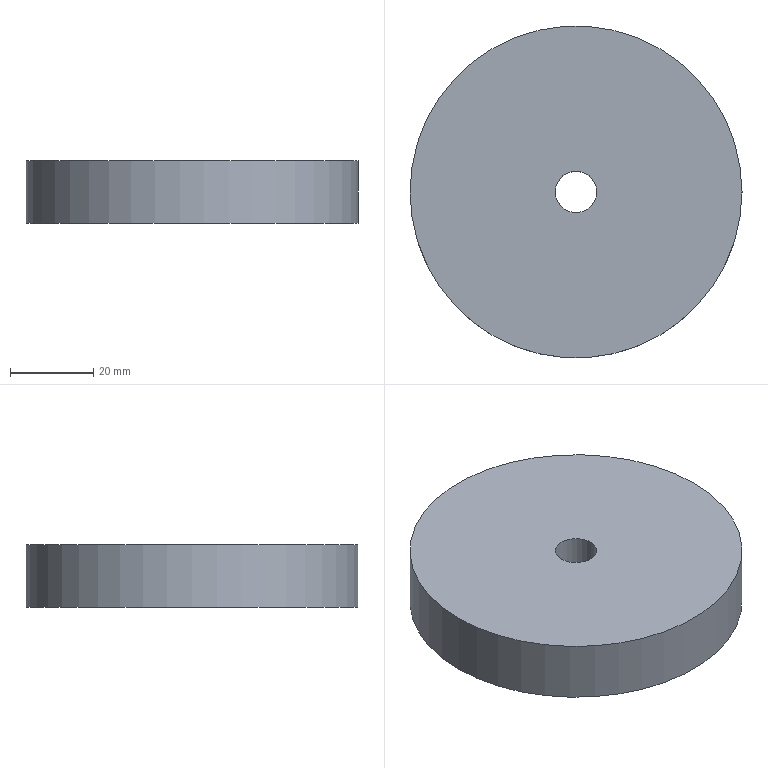Component | NX | CH3404_10-7 | 1 solid | 4 faces | box 80 x 80 x 15 mm | volume 74220 mm3 | cylinder 2 | plane 2 | commonest cylinder face diameters 80 x1 10 x1
STEP:
#1=CARTESIAN_POINT('',(0.,0.,0.));
#2=DIRECTION('',(0.,0.,1.));
#3=DIRECTION('',(1.,0.,0.));
#4=AXIS2_PLACEMENT_3D('',#1,#2,#3);
#5=CARTESIAN_POINT('',(40.,0.,202.));
#6=VERTEX_POINT('',#5);
#7=CARTESIAN_POINT('',(0.,0.,202.));
#8=DIRECTION('',(0.,0.,1.));
#9=DIRECTION('',(1.,0.,0.));
#10=AXIS2_PLACEMENT_3D('',#7,#8,#9);
#11=CIRCLE('',#10,40.);
#12=CARTESIAN_POINT('',(0.,0.,202.));
#13=DIRECTION('',(0.,0.,-1.));
#14=DIRECTION('',(-1.,0.,0.));
#15=AXIS2_PLACEMENT_3D('',#12,#13,#14);
#16=CYLINDRICAL_SURFACE('',#15,40.);
#17=CARTESIAN_POINT('',(9.425,0.));
#18=DIRECTION('',(-1.,0.));
#19=VECTOR('',#18,1.);
#20=LINE('',#17,#19);
#21=(GEOMETRIC_REPRESENTATION_CONTEXT(2)PARAMETRIC_REPRESENTATION_CONTEXT()REPRESENTATION_CONTEXT('',''));
#22=DEFINITIONAL_REPRESENTATION('',(#20),#21);
#23=PCURVE('',#16,#22);
#24=CARTESIAN_POINT('',(0.,0.,202.));
#25=DIRECTION('',(0.,0.,1.));
#26=DIRECTION('',(1.,0.,0.));
#27=AXIS2_PLACEMENT_3D('',#24,#25,#26);
#28=PLANE('',#27);
#29=CARTESIAN_POINT('',(0.,0.));
#30=DIRECTION('',(1.,0.));
#31=AXIS2_PLACEMENT_2D('',#29,#30);
#32=CIRCLE('',#31,40.);
#33=(GEOMETRIC_REPRESENTATION_CONTEXT(2)PARAMETRIC_REPRESENTATION_CONTEXT()REPRESENTATION_CONTEXT('',''));
#34=DEFINITIONAL_REPRESENTATION('',(#32),#33);
#35=PCURVE('',#28,#34);
#36=SURFACE_CURVE('',#11,(#23,#35),.PCURVE_S1.);
#37=EDGE_CURVE('',#6,#6,#36,.T.);
#38=ORIENTED_EDGE('',*,*,#37,.F.);
#39=CARTESIAN_POINT('',(40.,0.,187.));
#40=VERTEX_POINT('',#39);
#41=CARTESIAN_POINT('',(40.,0.,202.));
#42=CARTESIAN_POINT('',(40.,0.,187.));
#43=B_SPLINE_CURVE_WITH_KNOTS('',1,(#41,#42),.UNSPECIFIED.,.F.,.F.,(2,2),(0.,15.),.PIECEWISE_BEZIER_KNOTS.);
#44=CARTESIAN_POINT('',(9.425,0.));
#45=DIRECTION('',(0.,1.));
#46=VECTOR('',#45,1.);
#47=LINE('',#44,#46);
#48=(GEOMETRIC_REPRESENTATION_CONTEXT(2)PARAMETRIC_REPRESENTATION_CONTEXT()REPRESENTATION_CONTEXT('',''));
#49=DEFINITIONAL_REPRESENTATION('',(#47),#48);
#50=PCURVE('',#16,#49);
#51=CARTESIAN_POINT('',(3.142,0.));
#52=DIRECTION('',(0.,1.));
#53=VECTOR('',#52,1.);
#54=LINE('',#51,#53);
#55=(GEOMETRIC_REPRESENTATION_CONTEXT(2)PARAMETRIC_REPRESENTATION_CONTEXT()REPRESENTATION_CONTEXT('',''));
#56=DEFINITIONAL_REPRESENTATION('',(#54),#55);
#57=PCURVE('',#16,#56);
#58=SEAM_CURVE('',#43,(#50,#57),.PCURVE_S1.);
#59=EDGE_CURVE('',#6,#40,#58,.T.);
#60=ORIENTED_EDGE('',*,*,#59,.T.);
#61=CARTESIAN_POINT('',(0.,0.,187.));
#62=DIRECTION('',(0.,0.,1.));
#63=DIRECTION('',(1.,0.,0.));
#64=AXIS2_PLACEMENT_3D('',#61,#62,#63);
#65=CIRCLE('',#64,40.);
#66=CARTESIAN_POINT('',(9.425,15.));
#67=DIRECTION('',(-1.,0.));
#68=VECTOR('',#67,1.);
#69=LINE('',#66,#68);
#70=(GEOMETRIC_REPRESENTATION_CONTEXT(2)PARAMETRIC_REPRESENTATION_CONTEXT()REPRESENTATION_CONTEXT('',''));
#71=DEFINITIONAL_REPRESENTATION('',(#69),#70);
#72=PCURVE('',#16,#71);
#73=CARTESIAN_POINT('',(0.,0.,187.));
#74=DIRECTION('',(0.,0.,1.));
#75=DIRECTION('',(1.,0.,0.));
#76=AXIS2_PLACEMENT_3D('',#73,#74,#75);
#77=PLANE('',#76);
#78=CARTESIAN_POINT('',(0.,0.));
#79=DIRECTION('',(1.,0.));
#80=AXIS2_PLACEMENT_2D('',#78,#79);
#81=CIRCLE('',#80,40.);
#82=(GEOMETRIC_REPRESENTATION_CONTEXT(2)PARAMETRIC_REPRESENTATION_CONTEXT()REPRESENTATION_CONTEXT('',''));
#83=DEFINITIONAL_REPRESENTATION('',(#81),#82);
#84=PCURVE('',#77,#83);
#85=SURFACE_CURVE('',#65,(#72,#84),.PCURVE_S1.);
#86=EDGE_CURVE('',#40,#40,#85,.T.);
#87=ORIENTED_EDGE('',*,*,#86,.T.);
#88=ORIENTED_EDGE('',*,*,#59,.F.);
#89=EDGE_LOOP('',(#38,#60,#87,#88));
#90=FACE_BOUND('',#89,.T.);
#91=ADVANCED_FACE('',(#90),#16,.T.);
#92=CARTESIAN_POINT('',(5.,0.,202.));
#93=VERTEX_POINT('',#92);
#94=CARTESIAN_POINT('',(0.,0.,202.));
#95=DIRECTION('',(0.,0.,1.));
#96=DIRECTION('',(1.,0.,0.));
#97=AXIS2_PLACEMENT_3D('',#94,#95,#96);
#98=CIRCLE('',#97,5.);
#99=CARTESIAN_POINT('',(0.,0.,202.));
#100=DIRECTION('',(0.,0.,-1.));
#101=DIRECTION('',(-1.,0.,0.));
#102=AXIS2_PLACEMENT_3D('',#99,#100,#101);
#103=CYLINDRICAL_SURFACE('',#102,5.);
#104=CARTESIAN_POINT('',(9.425,0.));
#105=DIRECTION('',(-1.,0.));
#106=VECTOR('',#105,1.);
#107=LINE('',#104,#106);
#108=(GEOMETRIC_REPRESENTATION_CONTEXT(2)PARAMETRIC_REPRESENTATION_CONTEXT()REPRESENTATION_CONTEXT('',''));
#109=DEFINITIONAL_REPRESENTATION('',(#107),#108);
#110=PCURVE('',#103,#109);
#111=CARTESIAN_POINT('',(0.,0.));
#112=DIRECTION('',(1.,0.));
#113=AXIS2_PLACEMENT_2D('',#111,#112);
#114=CIRCLE('',#113,5.);
#115=(GEOMETRIC_REPRESENTATION_CONTEXT(2)PARAMETRIC_REPRESENTATION_CONTEXT()REPRESENTATION_CONTEXT('',''));
#116=DEFINITIONAL_REPRESENTATION('',(#114),#115);
#117=PCURVE('',#28,#116);
#118=SURFACE_CURVE('',#98,(#110,#117),.PCURVE_S1.);
#119=EDGE_CURVE('',#93,#93,#118,.T.);
#120=ORIENTED_EDGE('',*,*,#119,.F.);
#121=CARTESIAN_POINT('',(5.,0.,187.));
#122=VERTEX_POINT('',#121);
#123=CARTESIAN_POINT('',(5.,0.,202.));
#124=CARTESIAN_POINT('',(5.,0.,187.));
#125=B_SPLINE_CURVE_WITH_KNOTS('',1,(#123,#124),.UNSPECIFIED.,.F.,.F.,(2,2),(0.,15.),.PIECEWISE_BEZIER_KNOTS.);
#126=CARTESIAN_POINT('',(9.425,0.));
#127=DIRECTION('',(0.,1.));
#128=VECTOR('',#127,1.);
#129=LINE('',#126,#128);
#130=(GEOMETRIC_REPRESENTATION_CONTEXT(2)PARAMETRIC_REPRESENTATION_CONTEXT()REPRESENTATION_CONTEXT('',''));
#131=DEFINITIONAL_REPRESENTATION('',(#129),#130);
#132=PCURVE('',#103,#131);
#133=CARTESIAN_POINT('',(3.142,0.));
#134=DIRECTION('',(0.,1.));
#135=VECTOR('',#134,1.);
#136=LINE('',#133,#135);
#137=(GEOMETRIC_REPRESENTATION_CONTEXT(2)PARAMETRIC_REPRESENTATION_CONTEXT()REPRESENTATION_CONTEXT('',''));
#138=DEFINITIONAL_REPRESENTATION('',(#136),#137);
#139=PCURVE('',#103,#138);
#140=SEAM_CURVE('',#125,(#132,#139),.PCURVE_S1.);
#141=EDGE_CURVE('',#93,#122,#140,.T.);
#142=ORIENTED_EDGE('',*,*,#141,.T.);
#143=CARTESIAN_POINT('',(0.,0.,187.));
#144=DIRECTION('',(0.,0.,1.));
#145=DIRECTION('',(1.,0.,0.));
#146=AXIS2_PLACEMENT_3D('',#143,#144,#145);
#147=CIRCLE('',#146,5.);
#148=CARTESIAN_POINT('',(9.425,15.));
#149=DIRECTION('',(-1.,0.));
#150=VECTOR('',#149,1.);
#151=LINE('',#148,#150);
#152=(GEOMETRIC_REPRESENTATION_CONTEXT(2)PARAMETRIC_REPRESENTATION_CONTEXT()REPRESENTATION_CONTEXT('',''));
#153=DEFINITIONAL_REPRESENTATION('',(#151),#152);
#154=PCURVE('',#103,#153);
#155=CARTESIAN_POINT('',(0.,0.));
#156=DIRECTION('',(1.,0.));
#157=AXIS2_PLACEMENT_2D('',#155,#156);
#158=CIRCLE('',#157,5.);
#159=(GEOMETRIC_REPRESENTATION_CONTEXT(2)PARAMETRIC_REPRESENTATION_CONTEXT()REPRESENTATION_CONTEXT('',''));
#160=DEFINITIONAL_REPRESENTATION('',(#158),#159);
#161=PCURVE('',#77,#160);
#162=SURFACE_CURVE('',#147,(#154,#161),.PCURVE_S1.);
#163=EDGE_CURVE('',#122,#122,#162,.T.);
#164=ORIENTED_EDGE('',*,*,#163,.T.);
#165=ORIENTED_EDGE('',*,*,#141,.F.);
#166=EDGE_LOOP('',(#120,#142,#164,#165));
#167=FACE_BOUND('',#166,.F.);
#168=ADVANCED_FACE('',(#167),#103,.F.);
#169=ORIENTED_EDGE('',*,*,#37,.T.);
#170=EDGE_LOOP('',(#169));
#171=FACE_BOUND('',#170,.T.);
#172=ORIENTED_EDGE('',*,*,#119,.F.);
#173=EDGE_LOOP('',(#172));
#174=FACE_BOUND('',#173,.T.);
#175=ADVANCED_FACE('',(#171,#174),#28,.T.);
#176=ORIENTED_EDGE('',*,*,#86,.F.);
#177=EDGE_LOOP('',(#176));
#178=FACE_BOUND('',#177,.T.);
#179=ORIENTED_EDGE('',*,*,#163,.T.);
#180=EDGE_LOOP('',(#179));
#181=FACE_BOUND('',#180,.T.);
#182=ADVANCED_FACE('',(#178,#181),#77,.F.);
#183=CLOSED_SHELL('',(#91,#168,#175,#182));
#184=MANIFOLD_SOLID_BREP('',#183);
#185=(LENGTH_UNIT()NAMED_UNIT(*)SI_UNIT(.MILLI.,.METRE.));
#186=UNCERTAINTY_MEASURE_WITH_UNIT(LENGTH_MEASURE(0.00001),#185,'','');
#187=(NAMED_UNIT(*)PLANE_ANGLE_UNIT()SI_UNIT($,.RADIAN.));
#188=(NAMED_UNIT(*)SI_UNIT($,.STERADIAN.)SOLID_ANGLE_UNIT());
#189=(GEOMETRIC_REPRESENTATION_CONTEXT(3)GLOBAL_UNCERTAINTY_ASSIGNED_CONTEXT((#186))GLOBAL_UNIT_ASSIGNED_CONTEXT((#185,#187,#188))REPRESENTATION_CONTEXT('',''));
#190=ADVANCED_BREP_SHAPE_REPRESENTATION('',(#4,#184),#189);